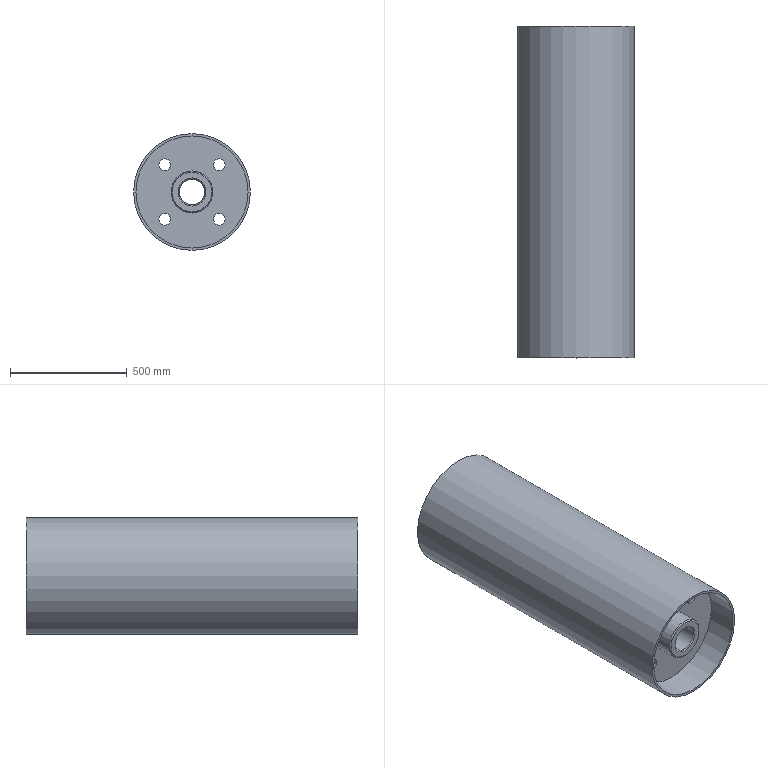Component | NX | ROLLER1 | 1 solid | 28 faces | volume 27659367 mm3 | cylinder 16 | plane 8 | cone 4 | commonest cylinder face diameters 50 x8 480 x3 110 x2 180 x2 500 x1